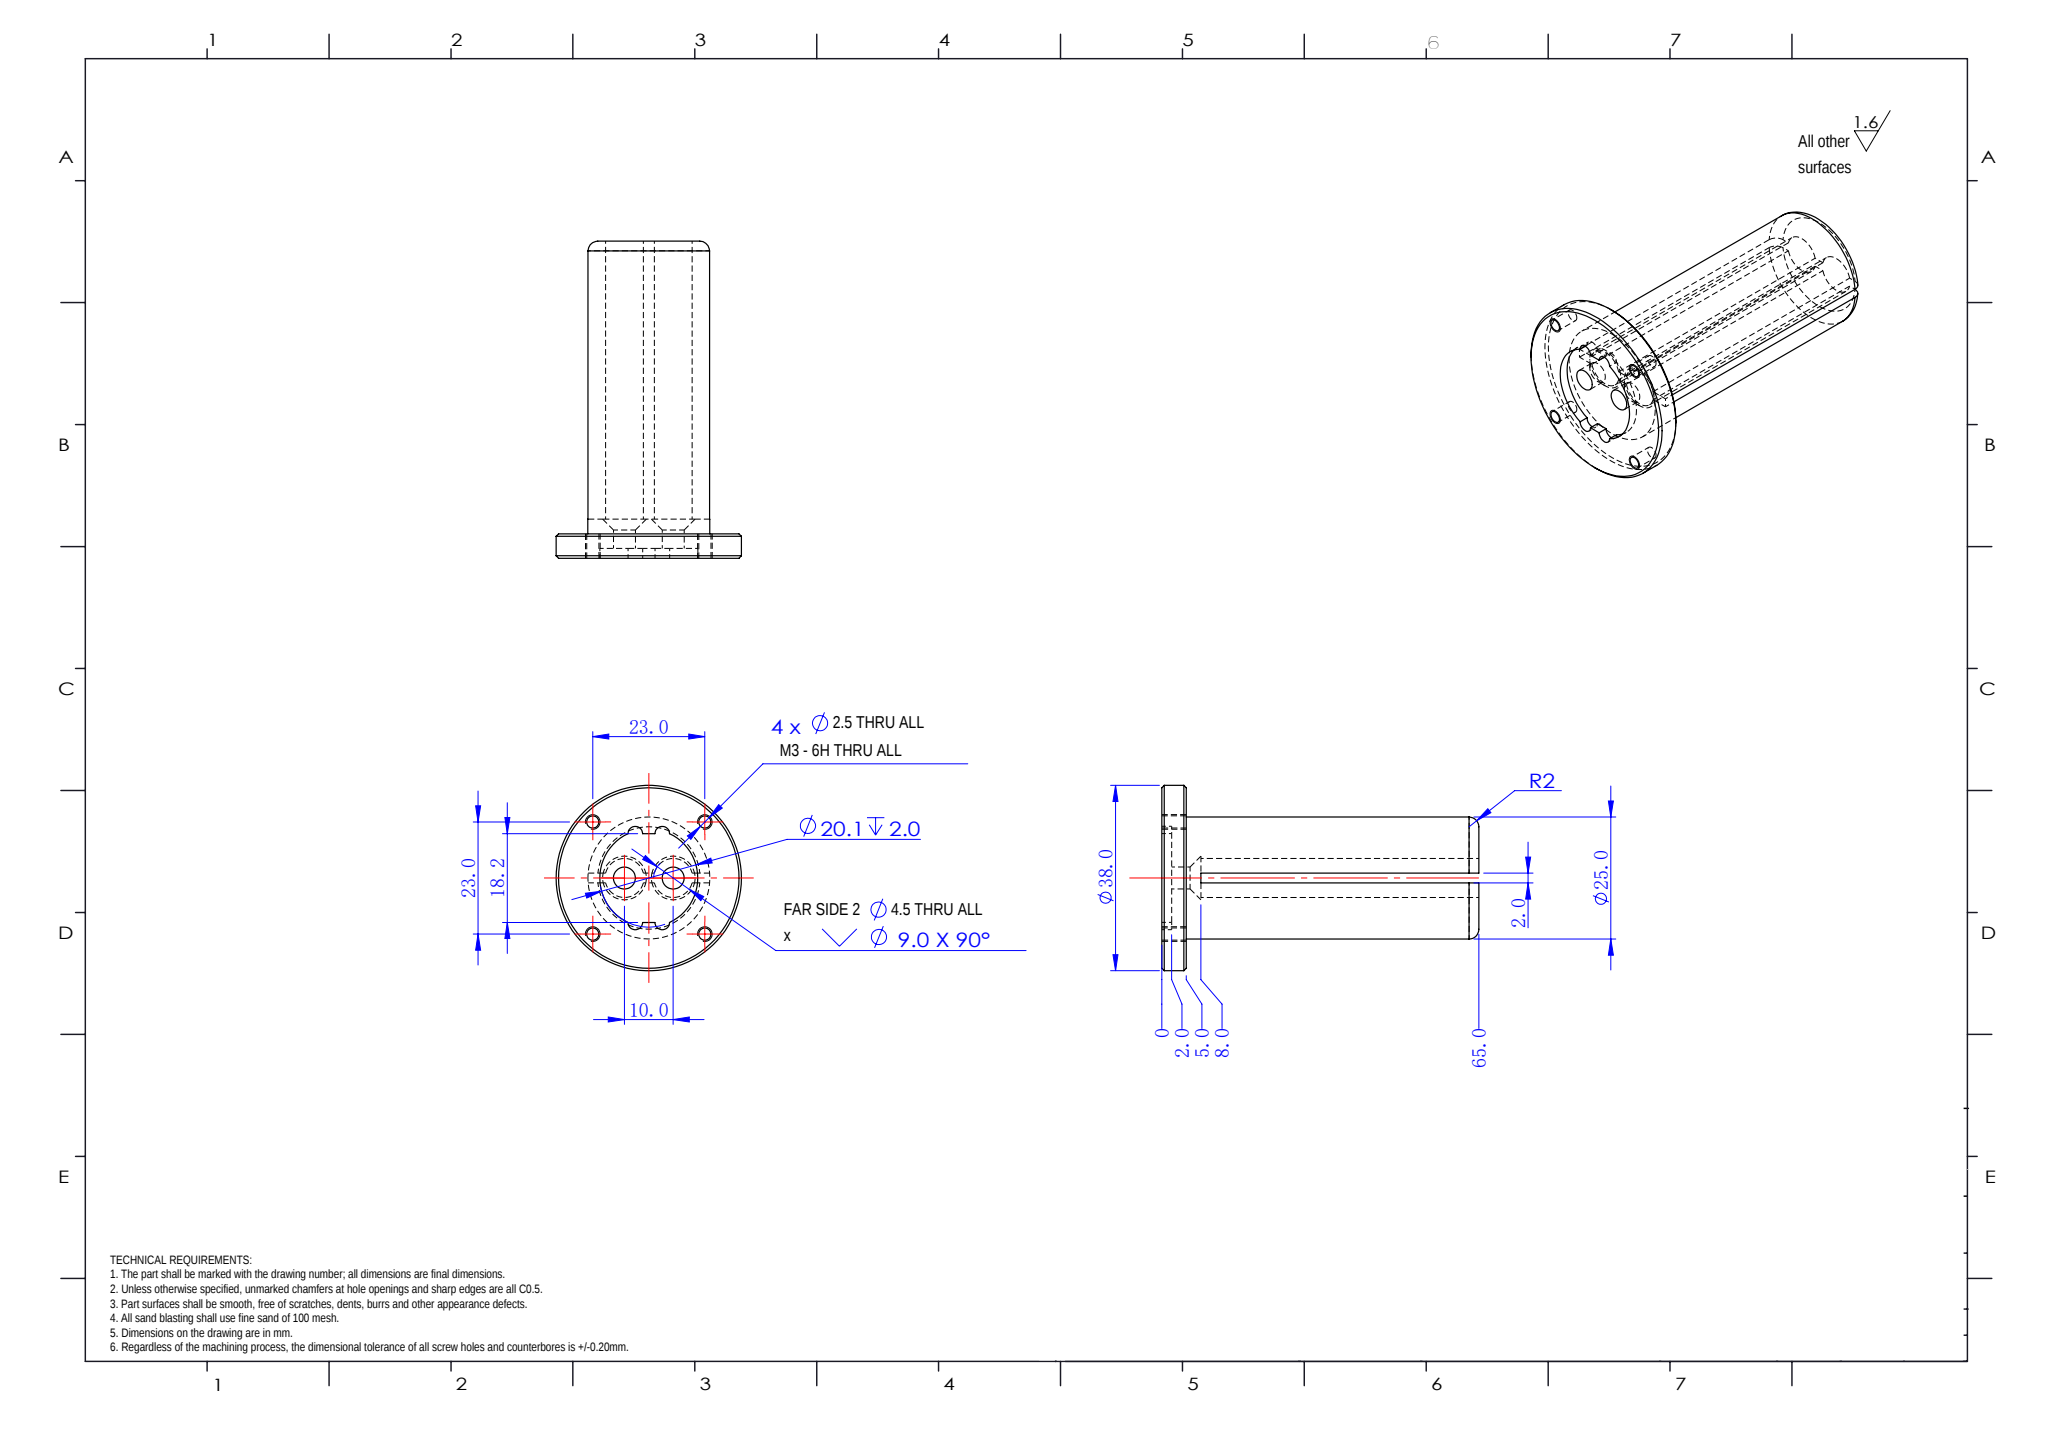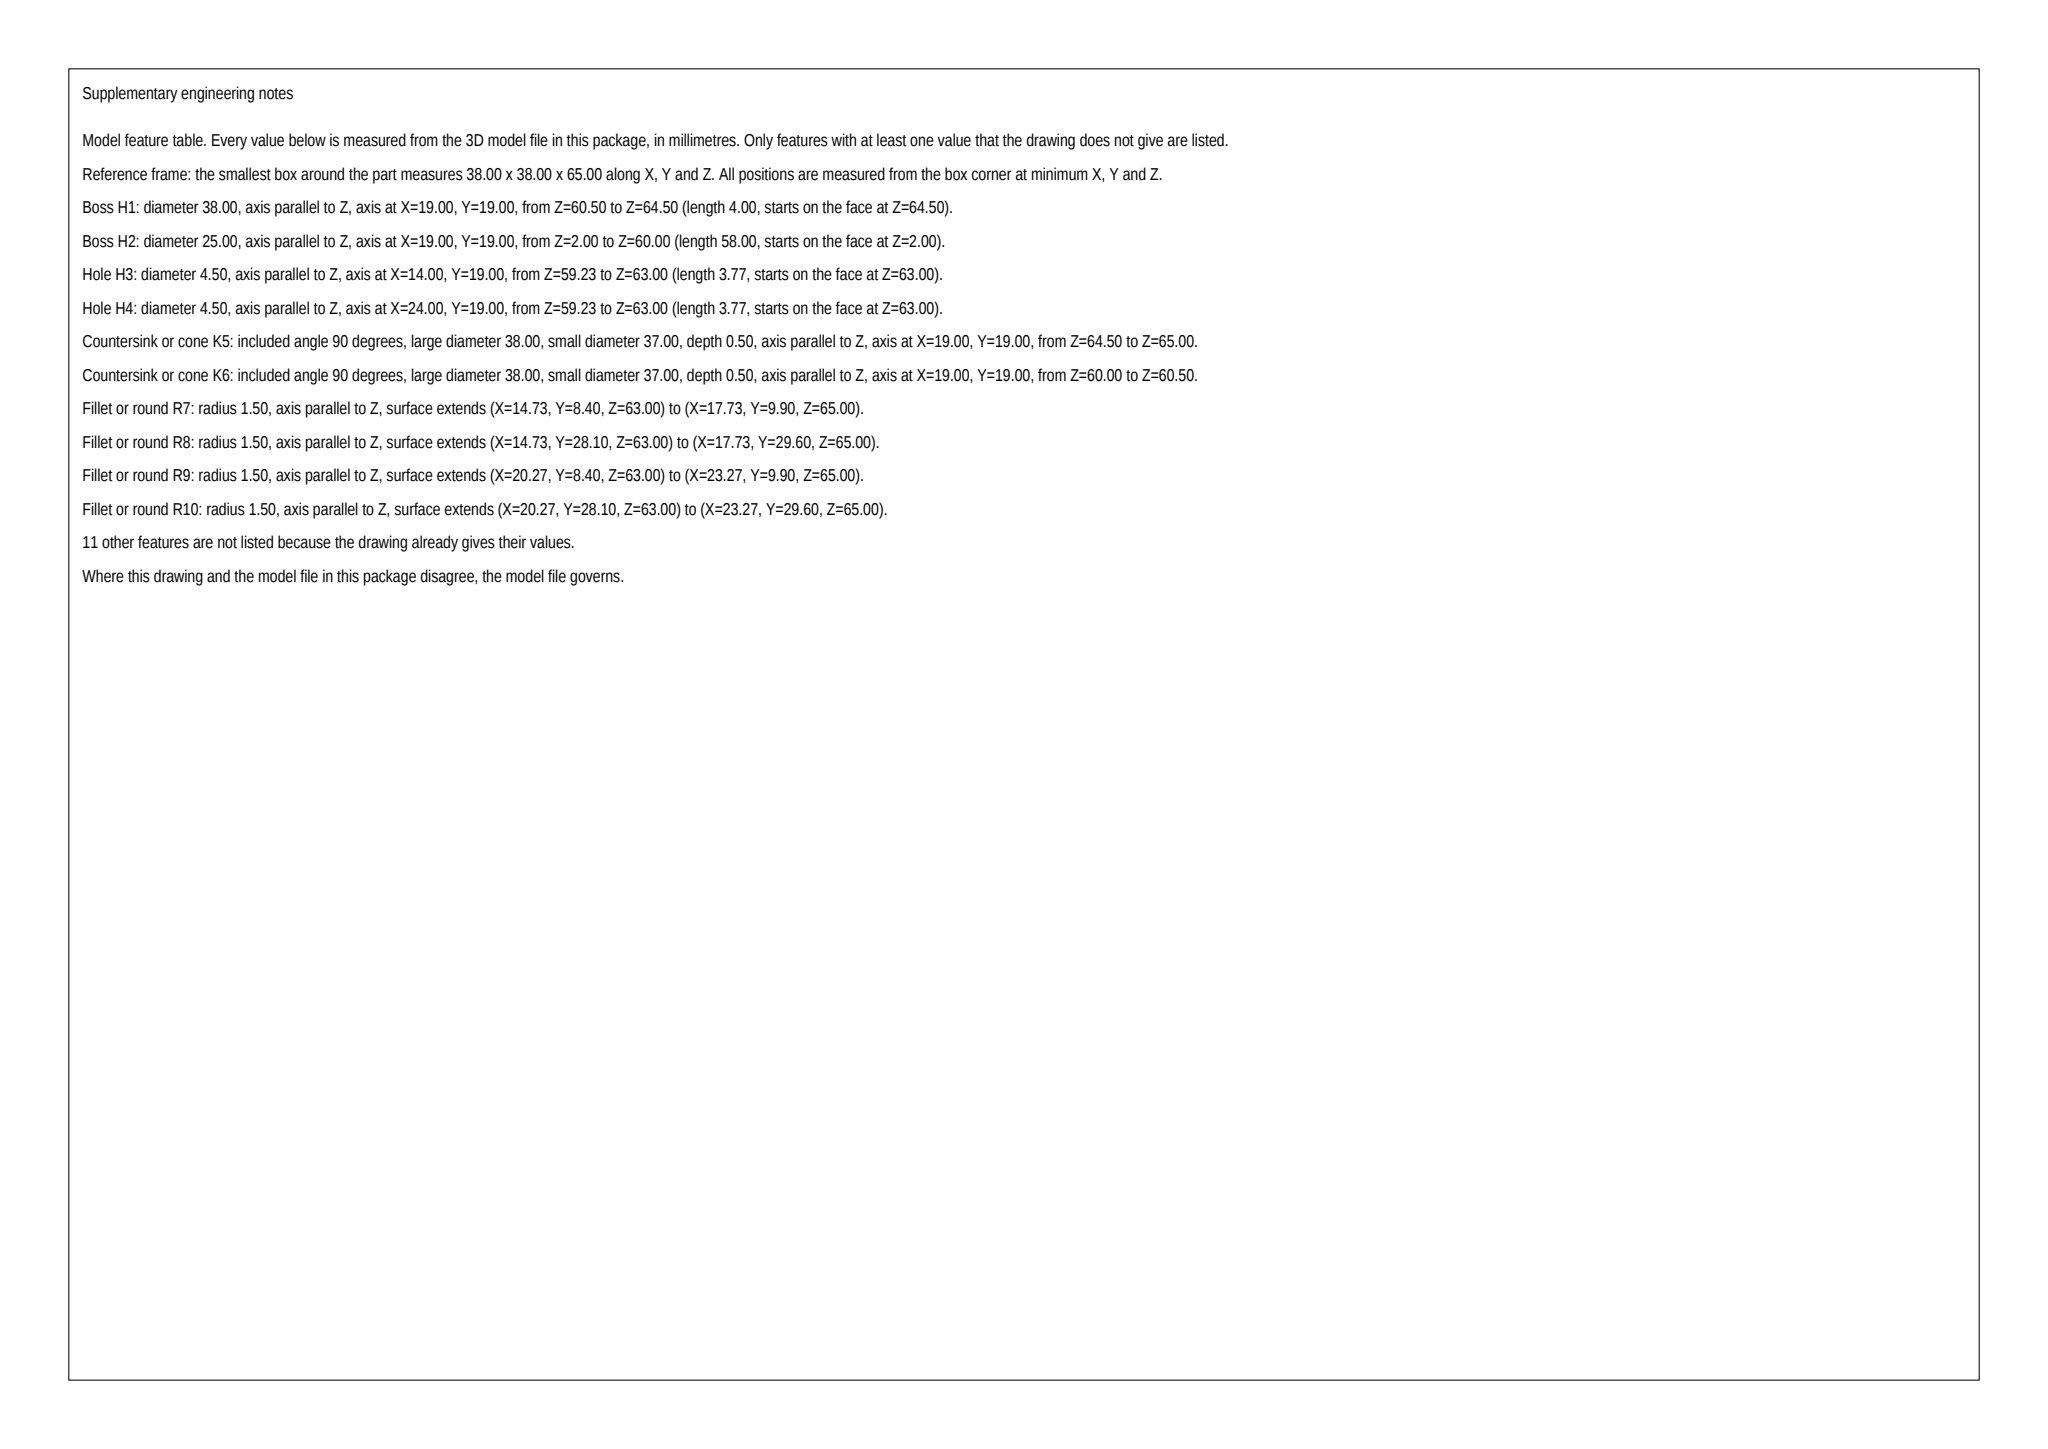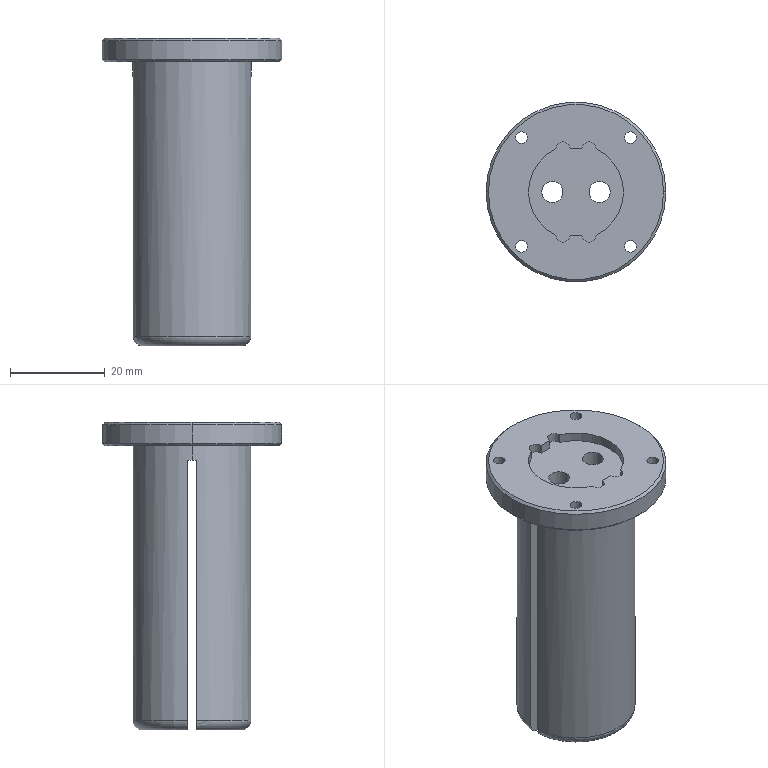Part | SolidWorks | mm | 1 solid | 57 faces | box 38 x 38 x 65 mm | volume 27236 mm3 | cylinder 27 | plane 20 | cone 8 | torus 2 | commonest cylinder face diameters 2.5 x8 4.5 x4 3 x4 8 x4 20.1 x3 25 x2 38 x2
build123d program:
from build123d import *

# Parameters (mm, degrees)
SKETCH1_R                                    = 19
BOSS_EXTRUDE1_DEPTH                          = 5
SKETCH2_R                                    = 12.5
BOSS_EXTRUDE2_DEPTH                          = 60
CUT_EXTRUDE1_DEPTH                           = 2
SKETCH6_R                                    = 1.5
CUT_EXTRUDE2_DEPTH                           = 2
SKETCH7_W                                    = 40
SKETCH7_H                                    = 2
CUT_EXTRUDE3_DEPTH                           = 57
M3_TAPPED_HOLE1_D                            = 2.5
SKETCH10_R                                   = 4
CUT_EXTRUDE4_DEPTH                           = 64.016
M4_HEXAGON_SOCKET_COUNTERSUNK_HEAD_S_2_COUNT = 2
M4_HEXAGON_SOCKET_COUNTERSUNK_HEAD_S_2_PITCH = 10
FILLET1_R                                    = 2
CHAMFER1_SIZE                                = 0.5


with BuildPart() as part:
    # Sketch1 → Boss-Extrude1 (new body)
    with BuildSketch(Plane.XY):
        Circle(SKETCH1_R)
    extrude(amount=BOSS_EXTRUDE1_DEPTH)

    # Sketch2 → Boss-Extrude2 (add)
    with BuildSketch(Plane(origin=(0, 0, 0), x_dir=(-1, 0, 0), z_dir=(0, 0, -1))):
        Circle(SKETCH2_R)
    extrude(amount=BOSS_EXTRUDE2_DEPTH)

    # Sketch5 → Cut-Extrude1 (cut)
    with BuildSketch(Plane.XY.offset(5)):
        with BuildLine():
            Line((-4.265, 9.1), (4.265, 9.1))
            ThreePointArc((4.265, 9.1), (10.05, 0), (4.265, -9.1))
            Line((4.265, -9.1), (-4.265, -9.1))
            ThreePointArc((-4.265, -9.1), (-10.05, 0), (-4.265, 9.1))
        make_face()
    extrude(amount=-CUT_EXTRUDE1_DEPTH, mode=Mode.SUBTRACT)

    # Sketch6 → Cut-Extrude2 (cut)
    with BuildSketch(Plane.XY.offset(5)):
        with Locations((-2.765, 9.1)):
            Circle(SKETCH6_R)
        with Locations((2.765, 9.1)):
            Circle(SKETCH6_R)
        with Locations((-2.765, -9.1)):
            Circle(SKETCH6_R)
        with Locations((2.765, -9.1)):
            Circle(SKETCH6_R)
    extrude(amount=-CUT_EXTRUDE2_DEPTH, mode=Mode.SUBTRACT)

    # Sketch7 → Cut-Extrude3 (cut)
    with BuildSketch(Plane(origin=(0, 0, -60), x_dir=(-1, 0, 0), z_dir=(0, 0, -1))):
        Rectangle(SKETCH7_W, SKETCH7_H)
    extrude(amount=-CUT_EXTRUDE3_DEPTH, mode=Mode.SUBTRACT)

    # M3 Tapped Hole1 (through all)
    with Locations(Plane.XY.offset(5)):
        with Locations((-11.49, 11.49), (11.49, 11.49), (-11.49, -11.49), (11.49, -11.49)):
            Hole(M3_TAPPED_HOLE1_D / 2)

    # Sketch10 → Cut-Extrude4 (cut, through all)
    with BuildSketch(Plane(origin=(0, 0, -3), x_dir=(-1, 0, 0), z_dir=(0, 0, -1))):
        with Locations((-5, 0)):
            Circle(SKETCH10_R)
        with Locations((5, 0)):
            Circle(SKETCH10_R)
    extrude(amount=CUT_EXTRUDE4_DEPTH, mode=Mode.SUBTRACT)

    # Sketch4 → M4 Hexagon Socket Countersunk Head Screw (revolve, cut)
    with BuildSketch(Plane(origin=(5, 0, -3), x_dir=(0, 1, 0), z_dir=(1, 0, 0))):
        Polygon((0, 0), (0, 8), (2.25, 8), (2.25, 2.23), (4.48, 0), align=None)
    m4_hexagon_socket_countersunk_head_screw = revolve(axis=Axis((5, 0, -9.35), (0, 0, 1)), mode=Mode.SUBTRACT)

    # M4 Hexagon Socket Countersunk Head S 2: M4 Hexagon Socket Countersunk Head Screw ×2
    with Locations(*[(-i * M4_HEXAGON_SOCKET_COUNTERSUNK_HEAD_S_2_PITCH, 0, 0) for i in range(1, M4_HEXAGON_SOCKET_COUNTERSUNK_HEAD_S_2_COUNT)]):
        add(m4_hexagon_socket_countersunk_head_screw, mode=Mode.SUBTRACT)

    # Fillet1
    fillet1_edges = [part.edges().sort_by_distance(p)[0] for p in [
        (0, -12.5, -60),
        (0, 12.5, -60),
    ]]
    fillet(fillet1_edges, radius=FILLET1_R)

    # Chamfer1
    chamfer1_edges = [part.edges().sort_by_distance(p)[0] for p in [
        (-19, 0, 0),
        (-19, 0, 5),
    ]]
    chamfer(chamfer1_edges, length=CHAMFER1_SIZE)


solid = part.part